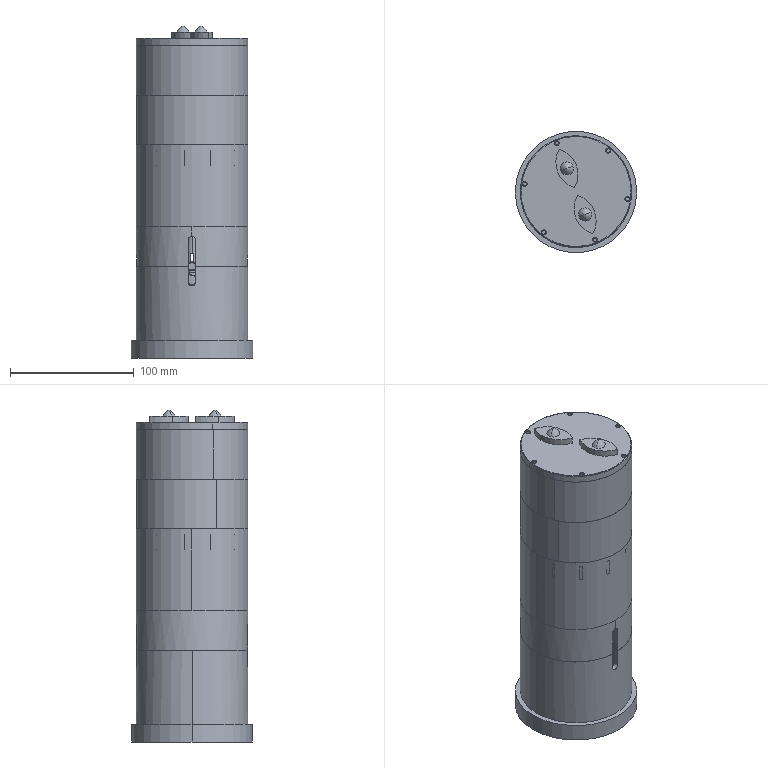Assembly | SolidWorks | mm | 21 component files | 21 solids | 793 faces | box 98 x 98 x 268.23 mm | volume 600372 mm3 | cylinder 394 | plane 251 | cone 76 | torus 72 | commonest cylinder face diameters 4 x43 3 x34 1.778 x32 8 x32 30.48 x28 2 x24 6 x22 86 x17
Bill of materials:
Cam2 | 1 |  | Thin-walled cylindrical cup whose open top rim is cut at an angle; flat floor with one small central through hole.
g | 1 |  | T-shaped body: a horizontal cylinder with chamfered ends meets a vertical cylindrical stem. The stem has a raised collar partway up and a small head at the top with radial lugs, each with a cross hole.
g1 | 1 |  | Cylindrical cup with an outer flange at the base and a stepped, reduced-diameter lip at the open top. Two opposite vertical slots with rounded ends run down from the rim. The floor has a large central hole and four small holes in a square pattern.
g11 | 1 |  | Plain cylindrical cup with a stepped, reduced-diameter lip at the open top. The floor has a large central hole and four small holes in a square pattern.
g2 | 1 |  | Shallow cylindrical cup with a stepped, reduced-diameter lip at the top. Flat floor with a single central through hole.
GMotor | 2 |  | Boxy body with a square-section core between a larger square top plate and a smaller square bottom flange. The top plate has four corner holes and a raised square pad with concentric circular steps. A short cylindrical shaft sticks out of the centre. Rounded vertical columns sit at the body corners.
GMotorAxis | 1 |  | Solid cylinder (pin or rod) with small chamfers on both end edges.
GMotorAxis | 1 |  | Short solid cylinder, about as long as it is wide or slightly longer, with chamfers on both end edges. A shallow, narrow slot or flat runs lengthwise along one side, starting at one end face and stopping partway down the body, where it ends in a curved runout.
GMotorCover | 1 |  | Shallow round tray with a thin, outward-flared lip flange at the top. Two opposite round-ended vertical slots run down from the rim. The floor has a rounded-square cutout, four small holes around it and a tiny centre hole.
GMotorCover2 | 1 |  | Shallow round tray with a thin, outward-flared lip flange and no wall slots. The floor has a rounded-square cutout, four small holes, two larger round holes on opposite sides of the cutout and a tiny centre hole.
GRingCam | 2 |  | Thin-walled cylindrical cup with a steeply angled open top, much taller on one side. Flat floor with a central through hole.
GuideCover | 1 |  | Short cylindrical puck or cap with a closed top face and a small step/chamfer around the top edge. The top has a central counterbored through hole. Two opposite round-ended slots run up from the bottom edge.
GuideRod1 | 1 |  | Stepped cylindrical pin with a smaller-diameter spigot at one end and a larger main body. The other end is split by a slot into a fork with a transverse through hole across both tines. The ends are chamfered.
hex nuts, style 1-grades ab gb | 2 |  | Hexagonal prism with a plain cylindrical through-bore along its axis and chamfered corners on both end faces; overall form of a hex nut.
JawCover | 1 |  | Thin circular plate with six small through-holes spaced around the rim and two raised pads, each with a pointed dome or cone-shaped tip, placed off-center on one face.
plain washers-chamfered--normal series-a gb | 1 |  | Flat annular ring (plain washer form): a thin disc with a large central hole and a chamfer on the outer edge of one face.
SpringCover | 1 |  | Shallow round cup or pot shape: a cylindrical shell with a closed bottom, an open top, and a short hollow central boss with a through-hole in the floor.
spur gear_gb | 1 |  | Flat toothed wheel with 12 rounded, pointed, petal-like teeth around a solid hub and a plain round center bore; overall form of a simple spur-gear-like disc.
Mates:
1. concentric | g1-1 face at (-15.928, -1.7, 30) dir (0, 0, -1) r 45 | GMotor-1 face at (-15.928, -1.7, 16) dir (0, 0, -1) r 2.5
2. coincident | g1-1 face at (-60.928, -1.7, -22) dir (0, 0, 1) | GMotor-1 face at (-15.928, -1.7, -22) dir (0, 0, -1)
3. concentric | g1-1 face at (-27.928, 10.3, -15) dir (0, 0, -1) r 2 | GMotor-1 face at (-27.928, 10.3, -22) dir (0, 0, -1) r 0.889
4. concentric | g1-1 face at (-15.928, -1.7, 30) dir (0, 0, -1) r 45 | GMotorCover-2 face at (-15.928, -1.7, 13) dir (0, 0, -1) r 40.5
5. parallel | GMotor-1 face at (1.572, -19.2, 11) dir (0, -1, 0) | GMotorCover-2 face at (-25.428, -15.2, 11) dir (0, 1, 0)
6. coincident | GMotor-1 face at (-15.928, -1.7, 11) dir (0, 0, 1) | GMotorCover-2 face at (-15.928, -1.7, 11) dir (0, 0, -1)
7. concentric | g1-1 face at (-15.928, -1.7, 30) dir (0, 0, -1) r 45 | GMotorAxis-1 face at (-15.928, -1.7, 27) dir (0, 0, -1) r 3
8. coincident | GMotor-1 face at (-15.928, -1.7, 11) dir (0, 0, 1) | GMotorAxis-1 face at (-15.928, -1.7, 11) dir (0, 0, -1)
9. concentric | GMotorCover-2 face at (-15.928, -1.7, 36) dir (0, 0, -1) r 39 | plain washers-chamfered--normal series-a gb-1 face at (-15.928, -1.7, 15.655) dir (0, 0, 1) r 5
10. coincident | plain washers-chamfered--normal series-a gb-1 face at (-15.928, -1.7, 16.655) dir (0, 0, 1) | hex nuts, style 1-grades ab gb-2 face at (-19.199, -10.339, 16.655) dir (0, 0, -1)
11. concentric | plain washers-chamfered--normal series-a gb-1 face at (-15.928, -1.7, 15.655) dir (0, 0, 1) r 5 | hex nuts, style 1-grades ab gb-2 face at (-15.928, -1.7, 16.655) dir (0, 0, 1) r 4.5
12. concentric | GMotorAxis-1 face at (-15.928, -1.7, 27) dir (0, 0, -1) r 3 | Cam2-1 face at (-15.928, -1.7, 35.655) dir (0, 0, -1) r 21
13. coincident | plain washers-chamfered--normal series-a gb-1 face at (-15.928, -1.7, 15.655) dir (0, 0, -1) | Cam2-1 face at (-15.928, -1.7, 15.655) dir (0, 0, 1)
14. concentric | Cam2-1 face at (-15.928, -1.7, 35.655) dir (0, 0, -1) r 19 | GuideCover-1 face at (-15.928, -1.7, 66) dir (0, 0, -1) r 45
15. coincident | g1-1 face at (-15.928, -1.7, 30) dir (0, 0, 1) | GuideCover-1 face at (-15.928, -1.7, 30) dir (0, 0, -1)
16. concentric | g1-1 face at (-15.928, -1.7, 30) dir (0, 0, -1) r 45 | GuideRod1-1 face at (-15.928, -1.7, 32) dir (0, 0, 1) r 4
17. coincident | GuideCover-1 face at (-15.928, -1.7, 62) dir (0, 0, -1) | GuideRod1-1 face at (-15.928, -1.7, 62) dir (0, 0, 1)
18. parallel | GMotor-1 face at (-30.928, -16.7, -22) dir (-1, 0, 0) | GuideRod1-1 face at (-17.428, -14.7, 24) dir (1, 0, 0)
19. parallel | g1-1 face at (-13.137, -131.7, 14) dir (-1, 0, 0) | GuideCover-1 face at (-12.928, 88.3, 6) dir (-1, 0, 0)
20. concentric | GuideRod1-1 face at (-15.928, -1.7, 70) dir (0, 0, -1) r 3 | hex nuts, style 1-grades ab gb-3 face at (-15.928, -1.7, 64) dir (0, 0, 1) r 4.5
21. coincident | GuideCover-1 face at (-15.928, -1.7, 64) dir (0, 0, 1) | hex nuts, style 1-grades ab gb-3 face at (-10.637, 5.872, 64) dir (0, 0, -1)
22. concentric | g1-1 face at (-15.928, -1.7, 30) dir (0, 0, -1) r 45 | g11-1 face at (-15.928, -1.7, 128) dir (0, 0, -1) r 45
23. coincident | GuideCover-1 face at (-60.928, -1.7, 62) dir (0, 0, 1) | g11-1 face at (-15.928, -1.7, 62) dir (0, 0, -1)
24. lock | GuideCover-1 reference at (0, 0, 0) dir (1, 0, 0) | g11-1 reference at (0, 0, 0) dir (1, 0, 0)
25. concentric | g11-1 face at (-15.928, -1.7, 128) dir (0, 0, -1) r 45 | GMotor-2 face at (-15.928, -1.7, 114) dir (0, 0, -1) r 2.5
26. concentric | g11-1 face at (-27.928, 10.3, 83) dir (0, 0, -1) r 2 | GMotor-2 face at (-27.928, 10.3, 76) dir (0, 0, -1) r 0.889
27. coincident | g11-1 face at (-60.928, -1.7, 76) dir (0, 0, 1) | GMotor-2 face at (-15.928, -1.7, 76) dir (0, 0, -1)
28. concentric | g11-1 face at (-15.928, -1.7, 128) dir (0, 0, -1) r 45 | GMotorCover2-1 face at (-15.928, -1.7, 111) dir (0, 0, -1) r 40.5
29. parallel | GMotor-2 face at (1.572, 15.8, 109) dir (1, 0, 0) | GMotorCover2-1 face at (-2.428, 7.8, 109) dir (-1, 0, 0)
30. coincident | g11-1 edge at (-15.928, -1.7, 134) dir (0, 0, -1) r 43 | GMotorCover2-1 face at (-15.928, -1.7, 134) dir (0, 0, -1)
31. concentric | g11-1 face at (-15.928, -1.7, 128) dir (0, 0, -1) r 45 | spur gear_gb-7 face at (-15.928, -1.7, 98.3) dir (0, 0, 1) r 9.525
32. coincident | GMotorCover2-1 face at (-15.928, -1.7, 111) dir (0, 0, 1) | spur gear_gb-7 face at (-15.928, -1.7, 111) dir (0, 0, -1)
33. concentric | GMotorCover2-1 face at (-15.928, 18.8, 119) dir (0, 0, -1) r 3 | spur gear_gb-5 face at (-15.928, 18.8, 136.4) dir (0, 0, -1) r 9.525
34. coincident | GMotorCover2-1 face at (-15.928, -1.7, 111) dir (0, 0, 1) | spur gear_gb-5 face at (-15.928, 18.8, 111) dir (0, 0, -1)
35. concentric | GMotorCover2-1 face at (-15.928, -22.2, 119) dir (0, 0, -1) r 3 | spur gear_gb-6 face at (-15.928, -22.2, 98.3) dir (0, 0, 1) r 9.525
36. coincident | GMotorCover2-1 face at (-15.928, -1.7, 111) dir (0, 0, 1) | spur gear_gb-6 face at (-15.928, -22.2, 111) dir (0, 0, -1)
37. concentric | g11-1 face at (-15.928, -1.7, 128) dir (0, 0, -1) r 45 | GMotorAxis-2 face at (-15.928, -1.7, 117) dir (0, 0, -1) r 3
38. coincident | GMotor-2 face at (-6.428, -11.2, 109.3) dir (0, 0, 1) | GMotorAxis-2 face at (-15.928, -1.7, 109.3) dir (0, 0, -1)
39. gear | spur gear_gb-6 face at (-15.928, -22.2, 111) dir (0, 0, 1) r 30.161 | spur gear_gb-7 face at (-15.928, -1.7, 111) dir (0, 0, 1) r 30.161
40. gear | spur gear_gb-7 face at (-15.928, -1.7, 111) dir (0, 0, 1) r 30.161 | spur gear_gb-5 face at (-15.928, 18.8, 123.7) dir (0, 0, -1) r 30.161
41. lock | spur gear_gb-5 reference at (0, 0, 0) dir (1, 0, 0) | GRingCam-10 reference at (0, 0, 0) dir (1, 0, 0)
42. concentric | spur gear_gb-6 face at (-15.928, -22.2, 98.3) dir (0, 0, 1) r 9.525 | GRingCam-8 face at (-15.928, -22.2, 133) dir (0, 0, -1) r 18
43. coincident | spur gear_gb-6 face at (-15.928, -22.2, 123.7) dir (0, 0, 1) | GRingCam-8 face at (-15.928, -22.2, 117) dir (0, 0, -1)
44. lock | spur gear_gb-6 reference at (0, 0, 0) dir (1, 0, 0) | GRingCam-8 reference at (0, 0, 0) dir (1, 0, 0)
45. concentric | g11-1 face at (-15.928, -1.7, 128) dir (0, 0, -1) r 45 | g-1 face at (-15.928, -1.7, 199.035) dir (0, 0, -1) r 6
46. parallel | GMotor-2 face at (-0.928, -16.7, 76) dir (0, -1, 0) | g-1 face at (-15.928, -21.7, 129.035) dir (0, -1, 0)
47. concentric | g1-1 face at (-15.928, -1.7, 30) dir (0, 0, -1) r 45 | g2-1 face at (-15.928, -1.7, 128) dir (0, 0, 1) r 45
48. coincident | g11-1 face at (-15.928, -1.7, 128) dir (0, 0, 1) | g2-1 face at (-15.928, -1.7, 128) dir (0, 0, -1)
49. concentric | g2-1 face at (-15.928, -1.7, 128) dir (0, 0, 1) r 45 | SpringCover-2 face at (-15.928, -1.7, 168) dir (0, 0, 1) r 45
50. coincident | g2-1 face at (-15.928, -1.7, 168) dir (0, 0, 1) | SpringCover-2 face at (-15.928, -1.7, 168) dir (0, 0, -1)
51. concentric | SpringCover-2 face at (-15.928, -1.7, 168) dir (0, 0, 1) r 45 | JawCover-1 face at (-15.928, -1.7, 214) dir (0, 0, -1) r 45
52. coincident | SpringCover-2 face at (-15.928, -1.7, 208) dir (0, 0, 1) | JawCover-1 face at (-15.928, -1.7, 208) dir (0, 0, -1)